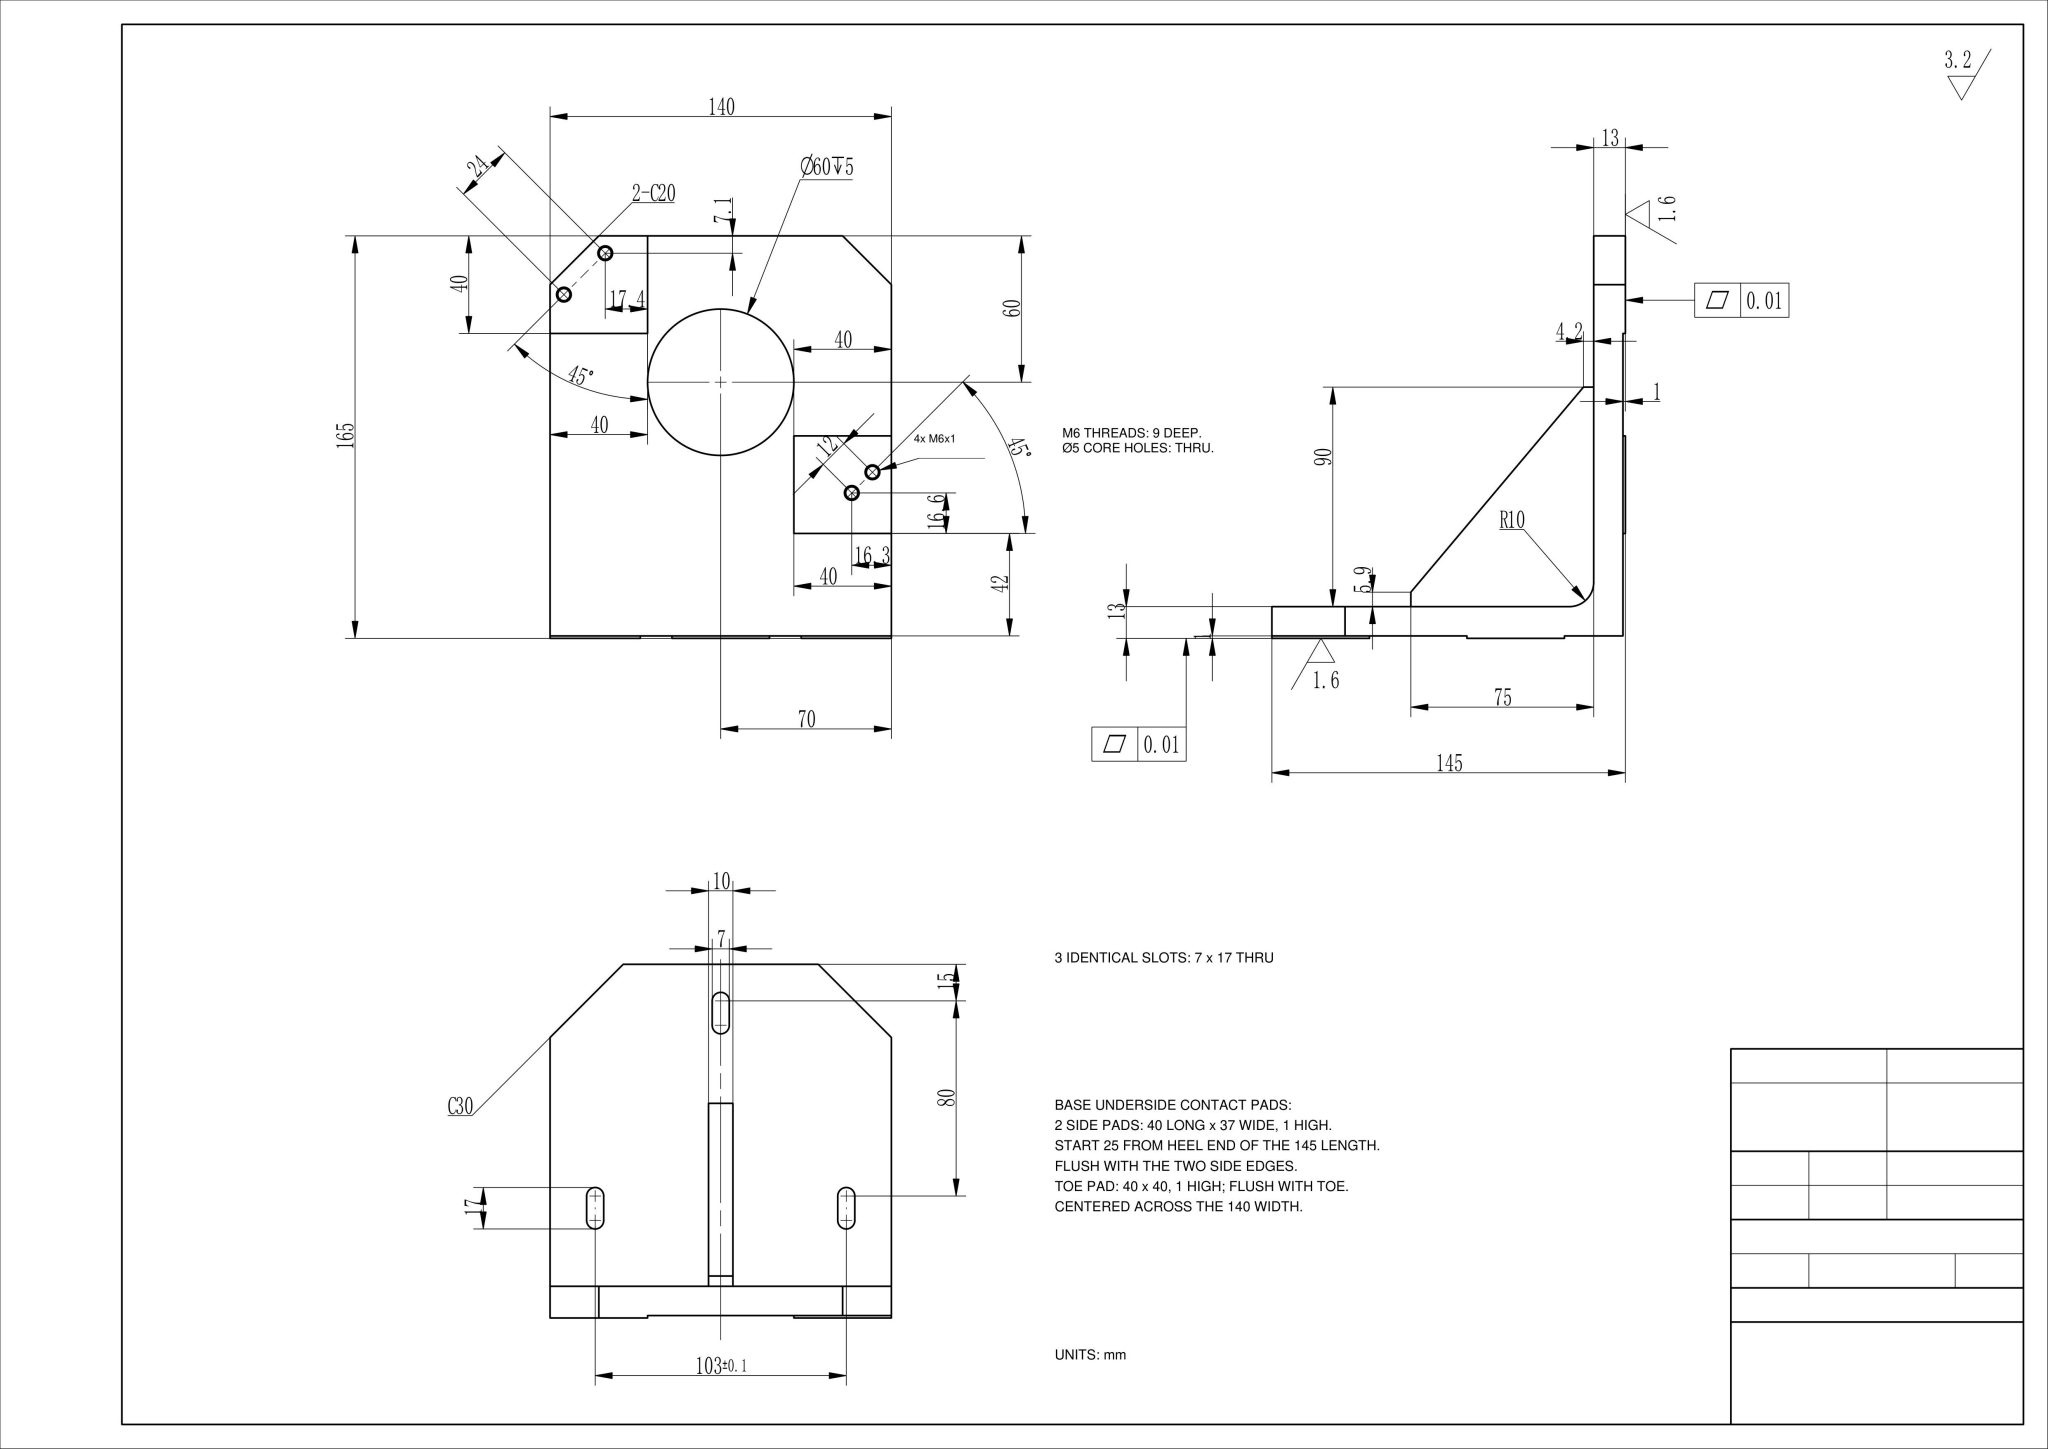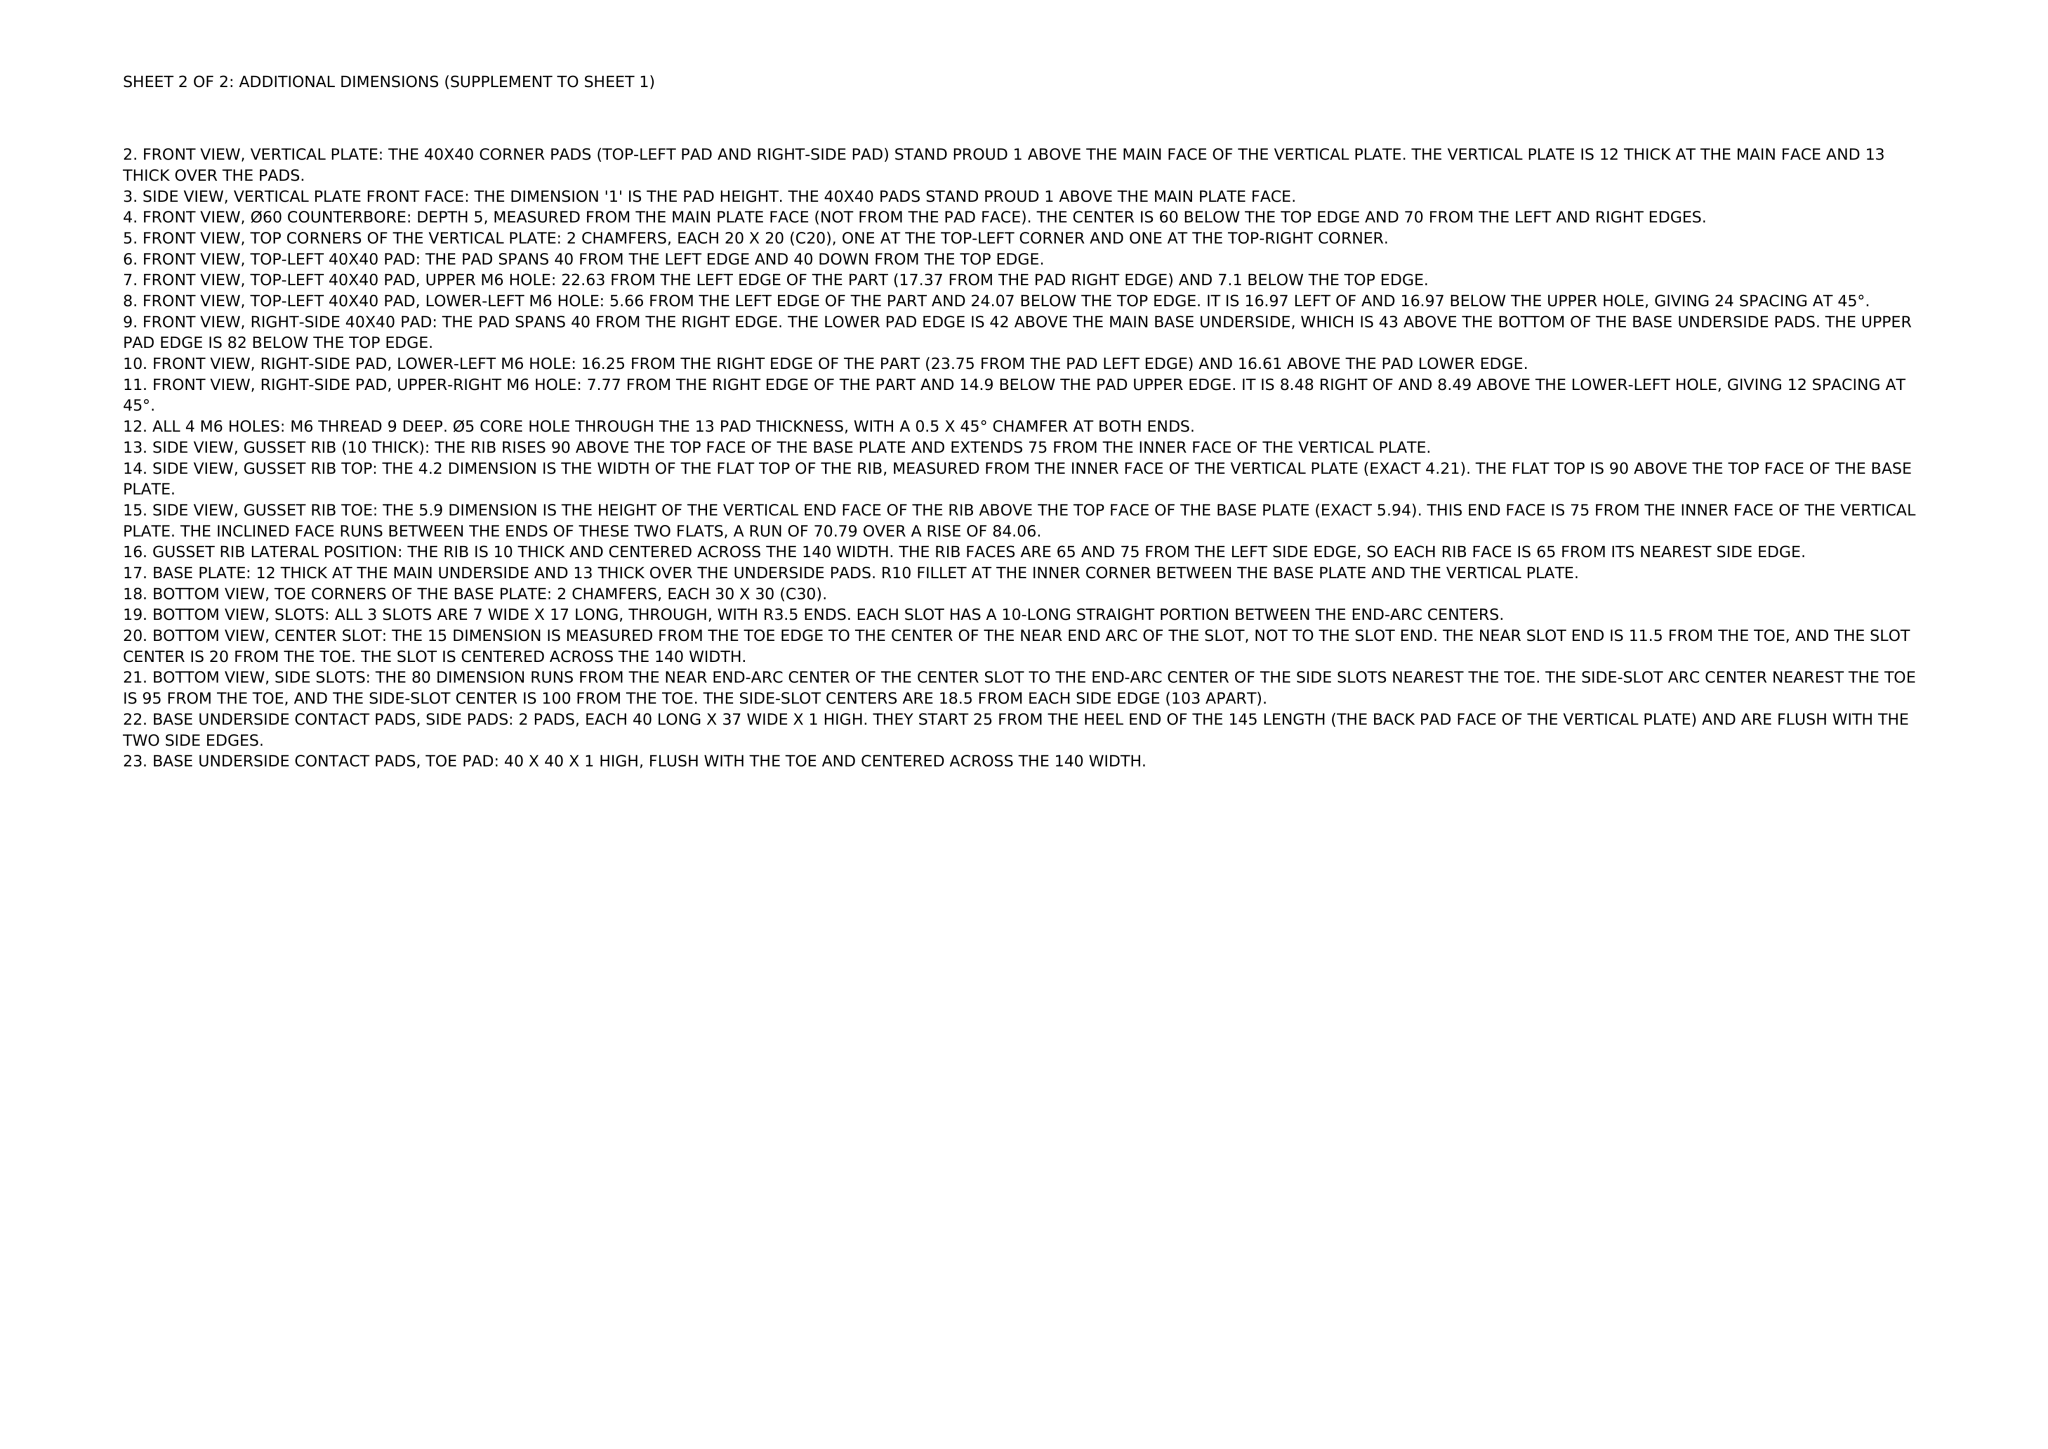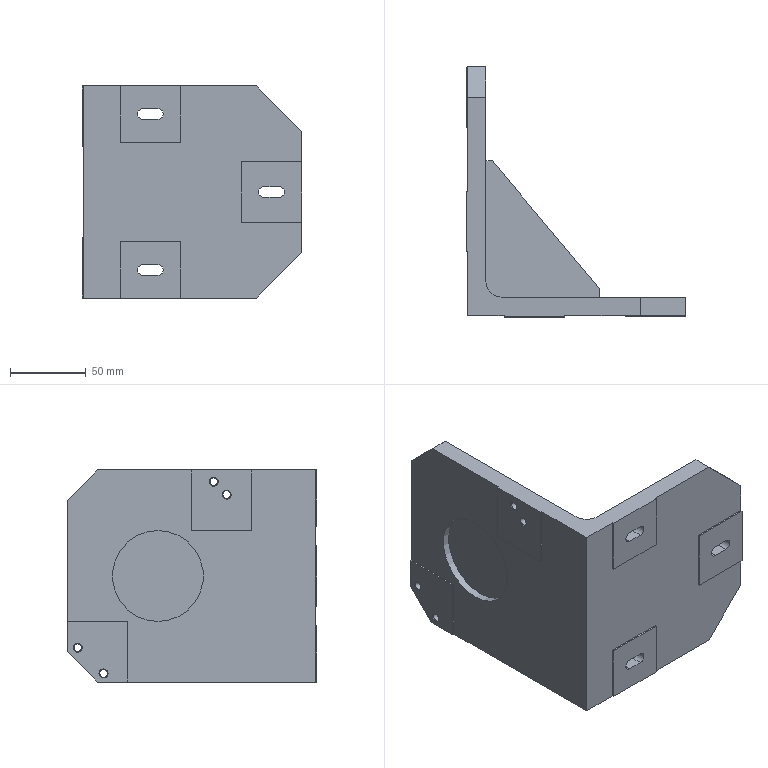Part | NX | mm | 1 solid | 64 faces | box 145 x 165 x 140 mm | volume 510370 mm3 | plane 43 | cylinder 13 | cone 8 | commonest cylinder face diameters 7 x6 5 x4 20 x2 60 x1